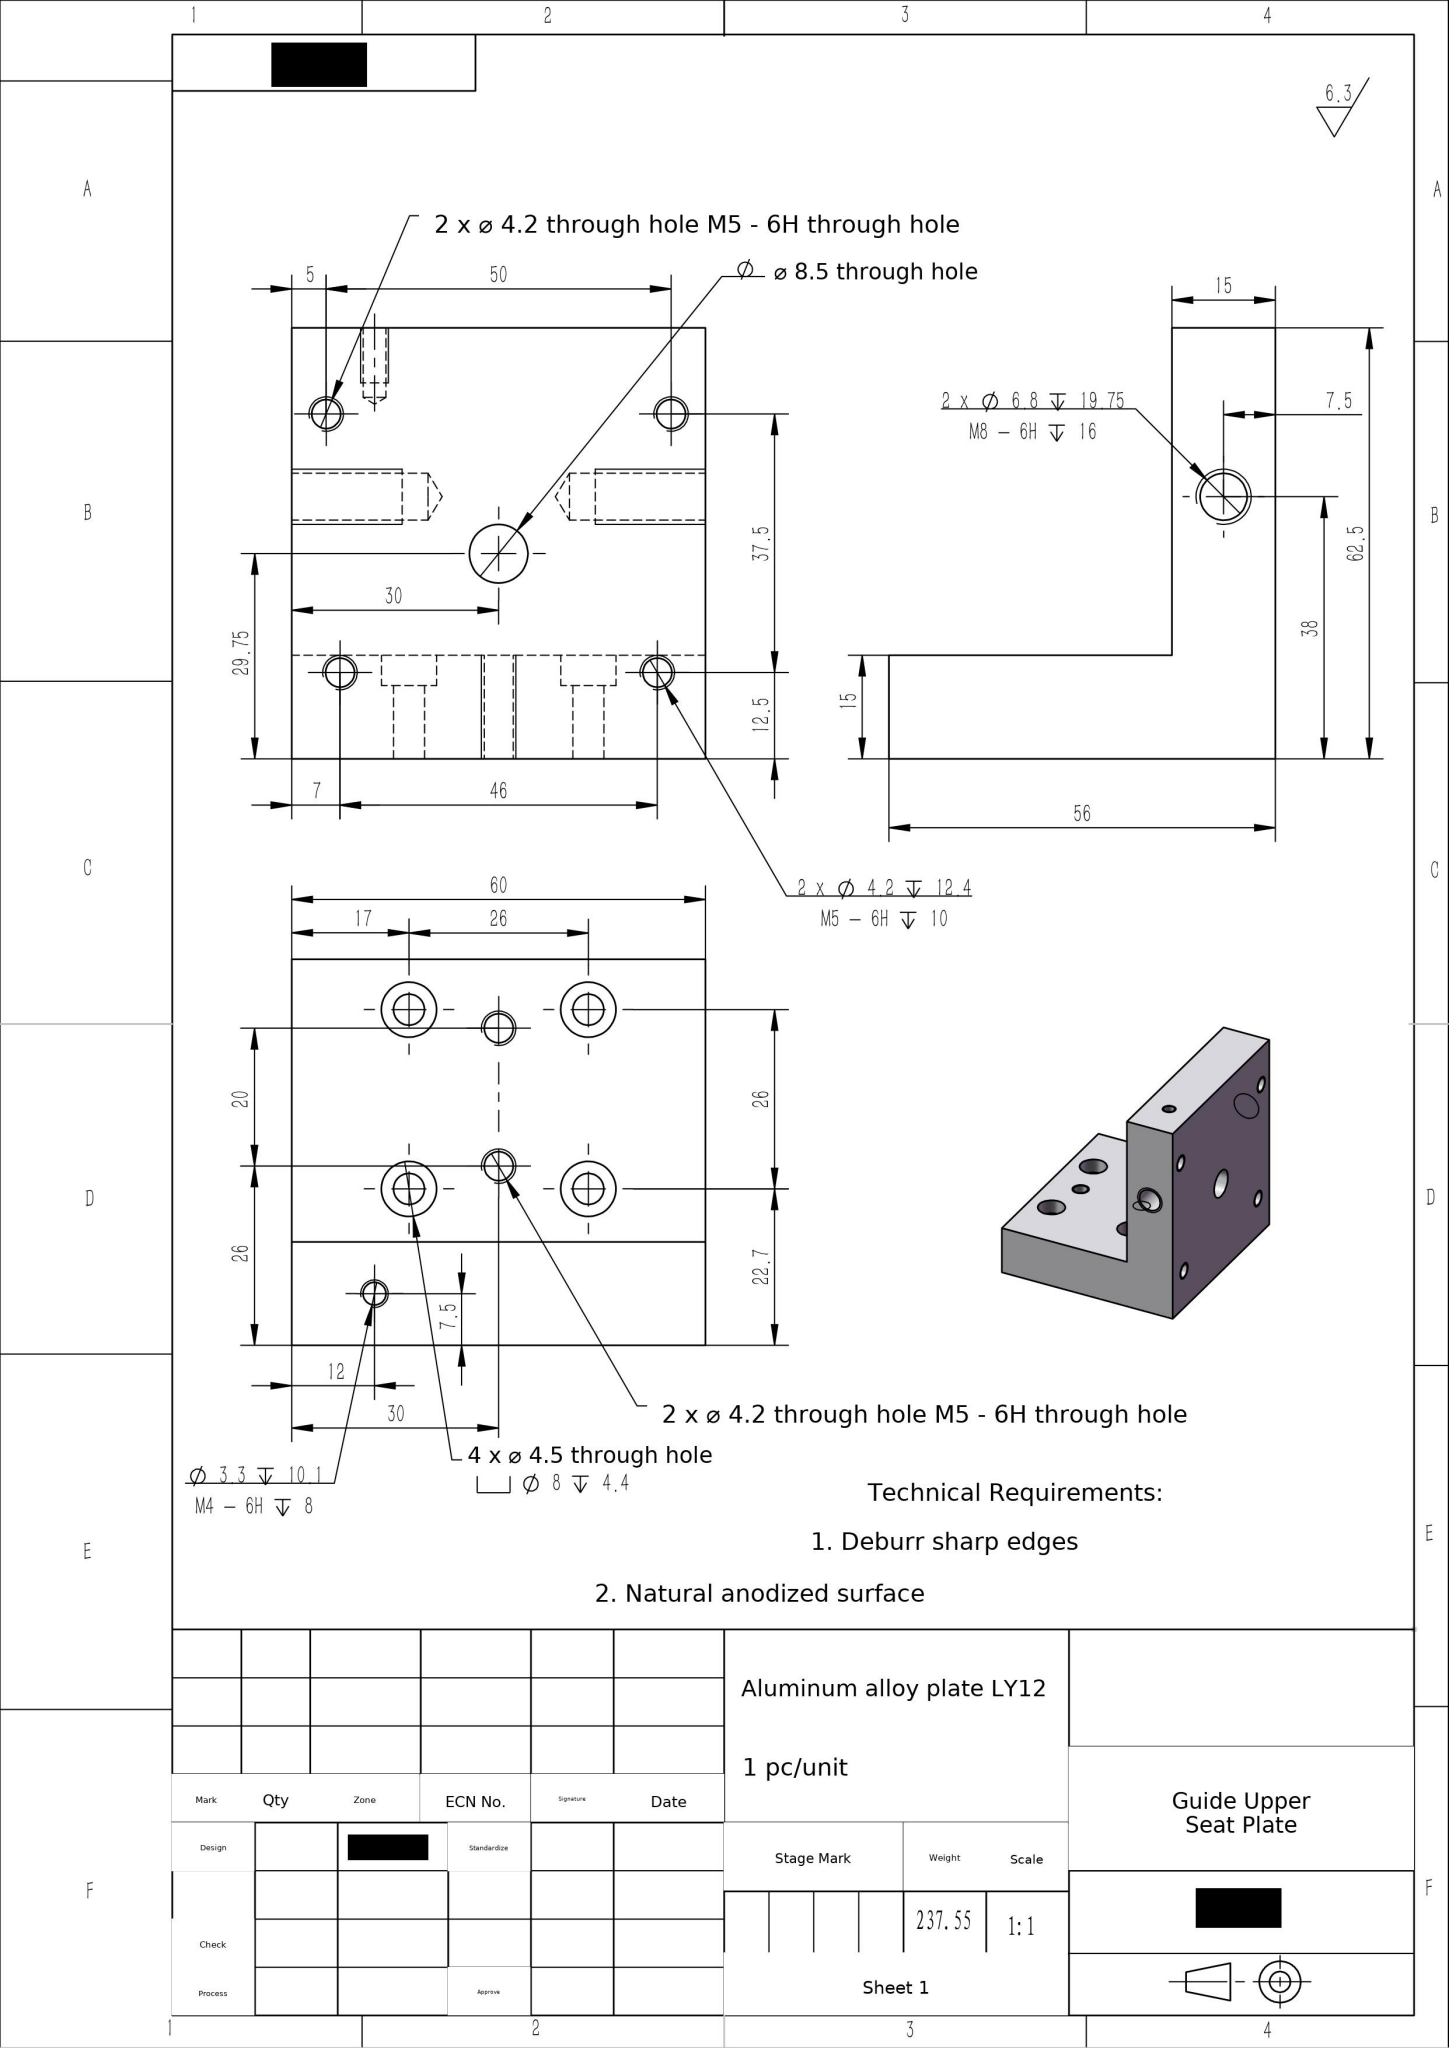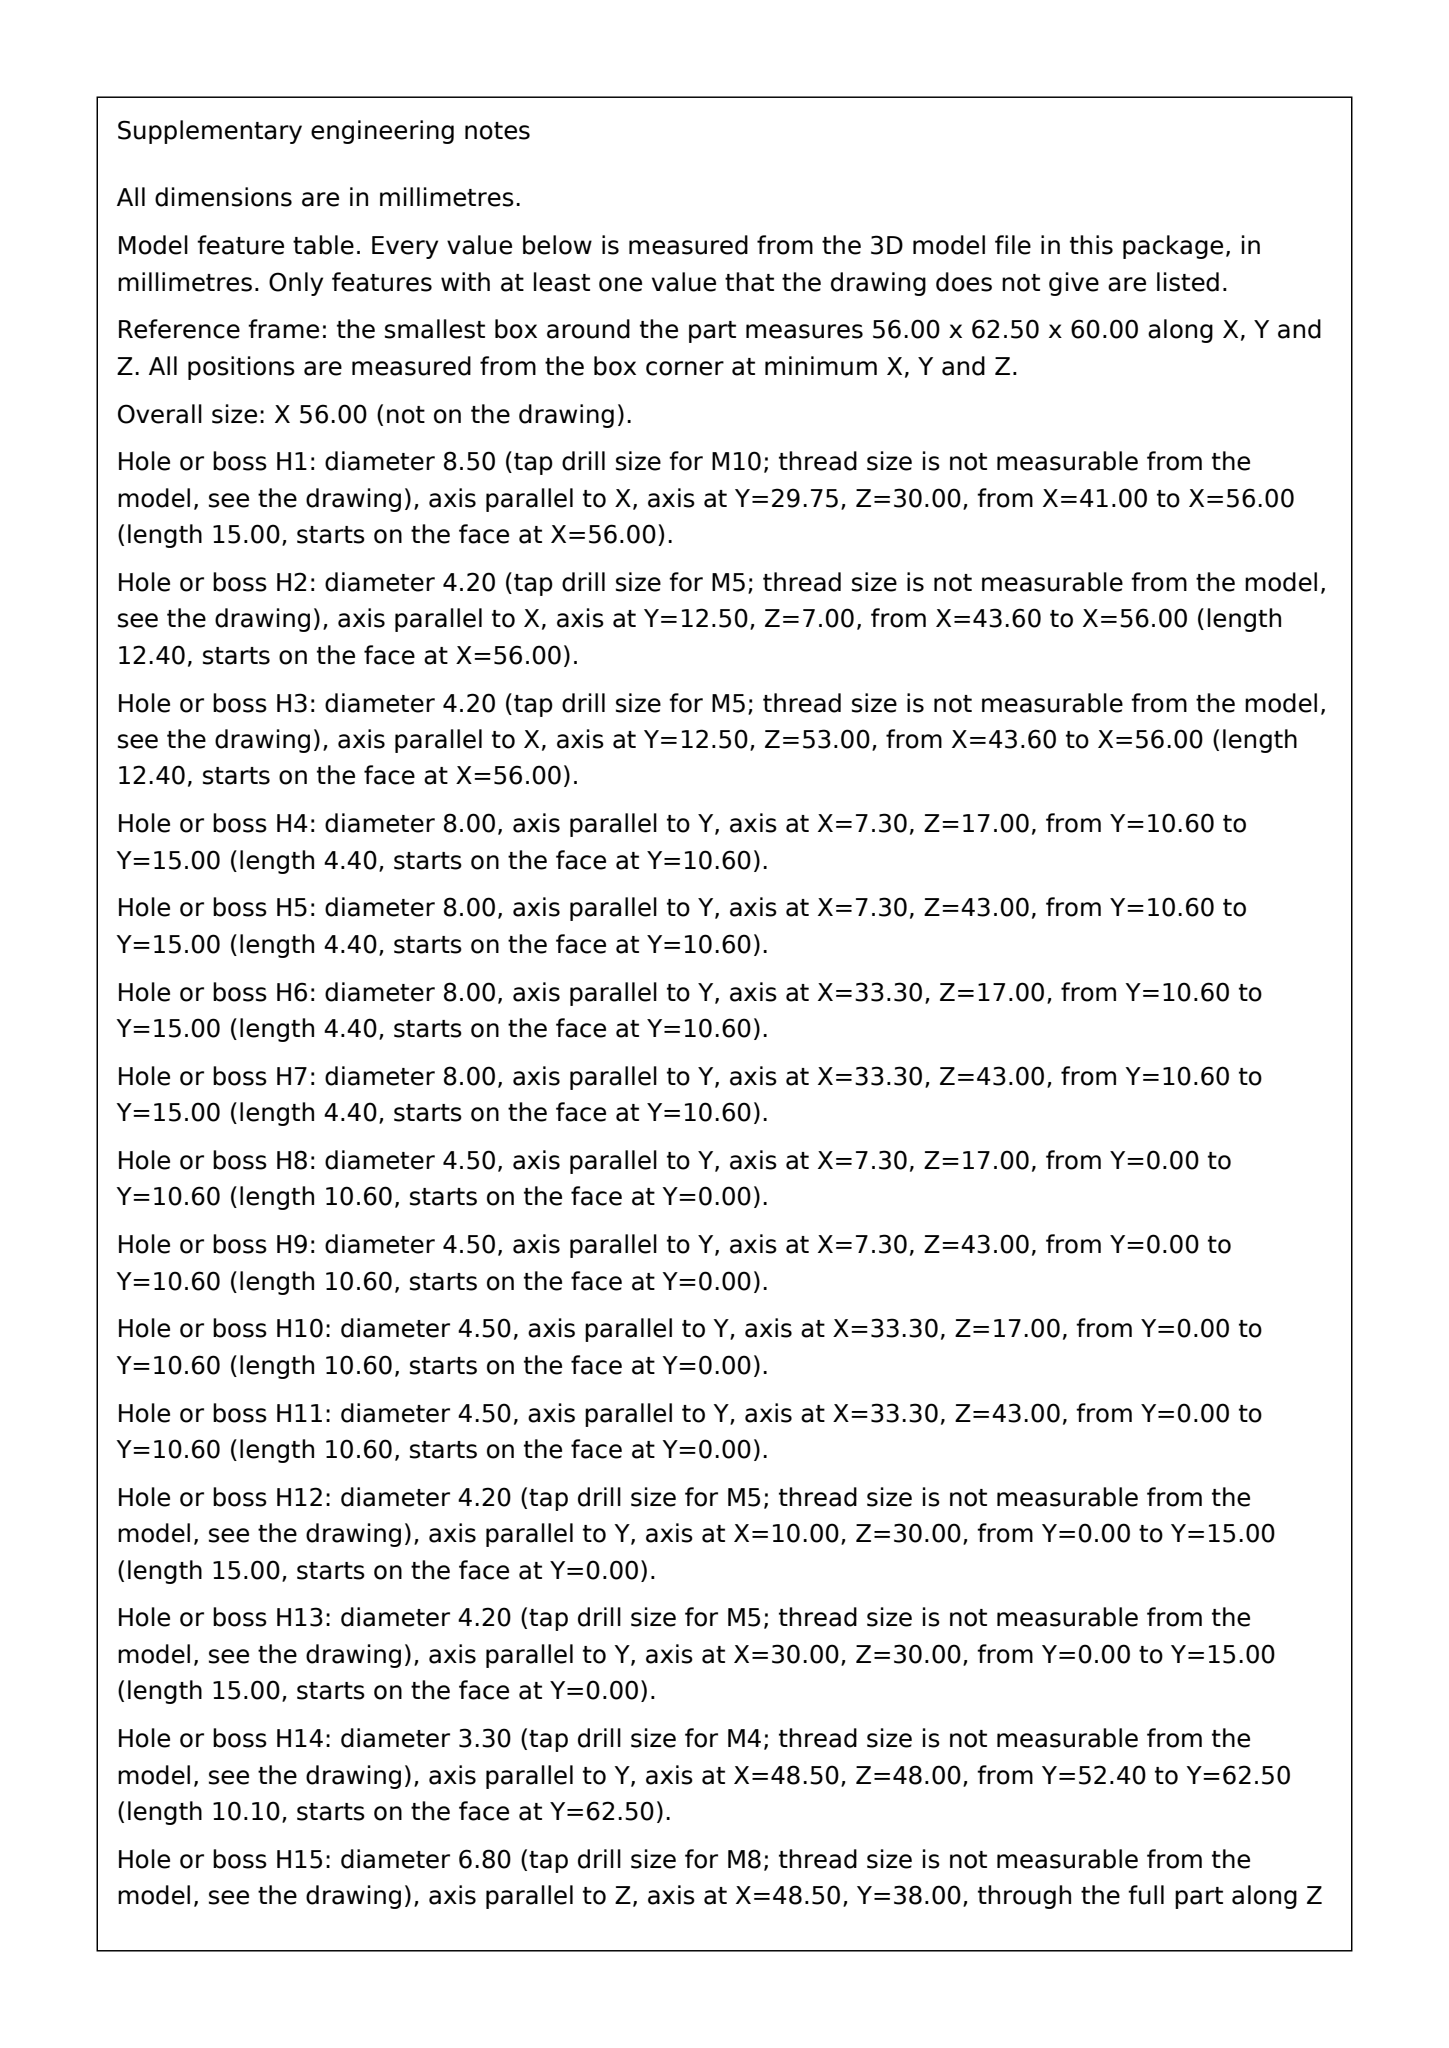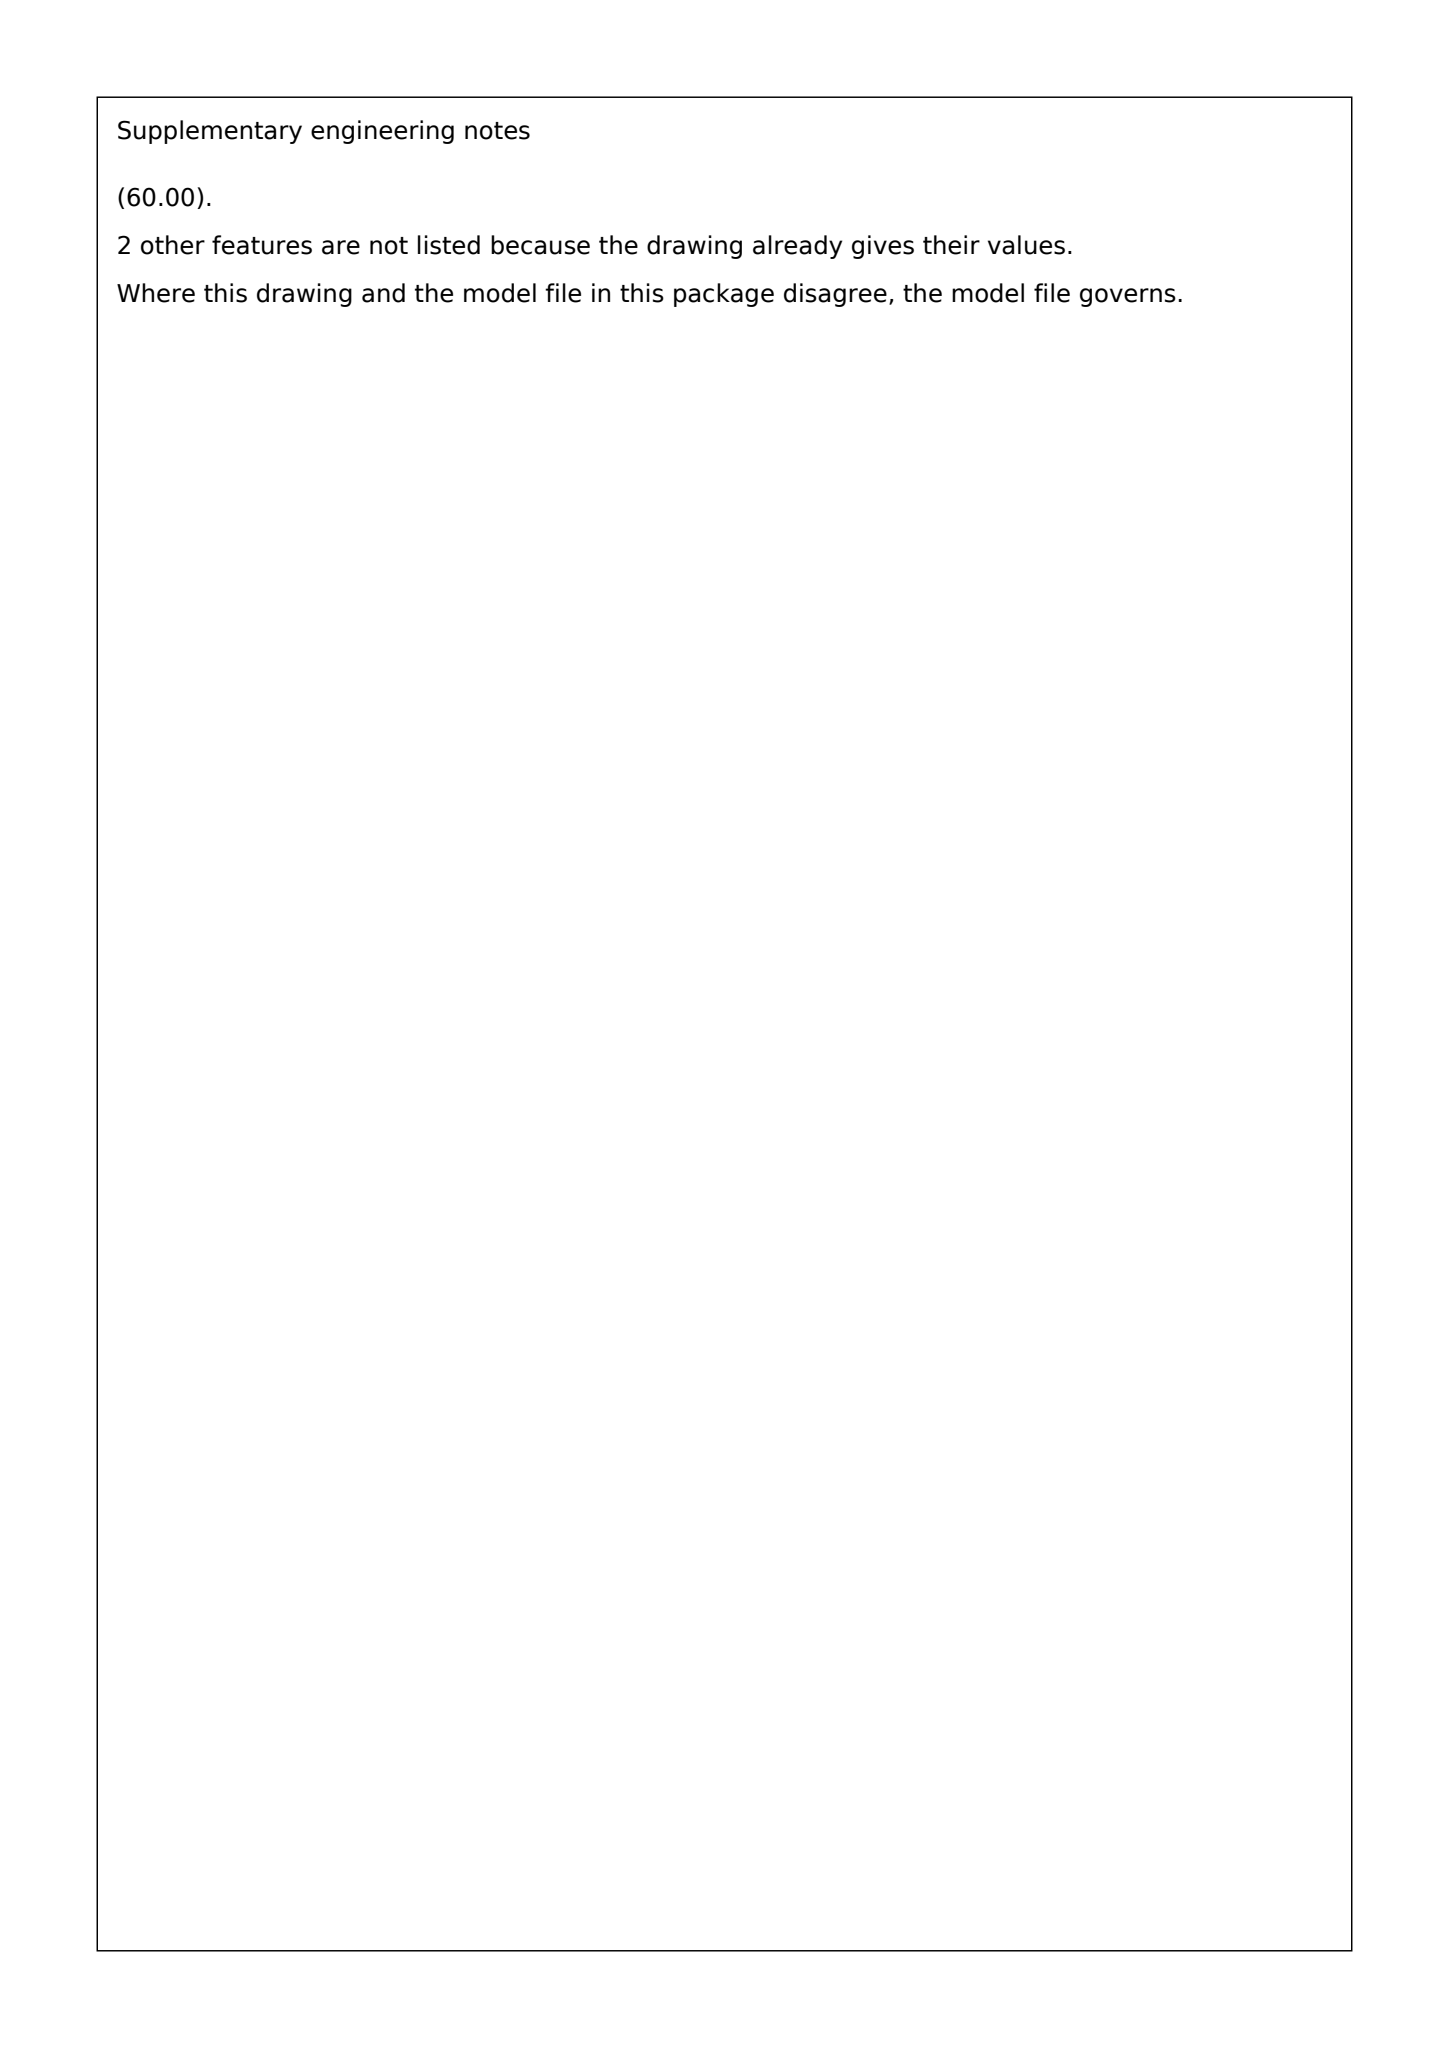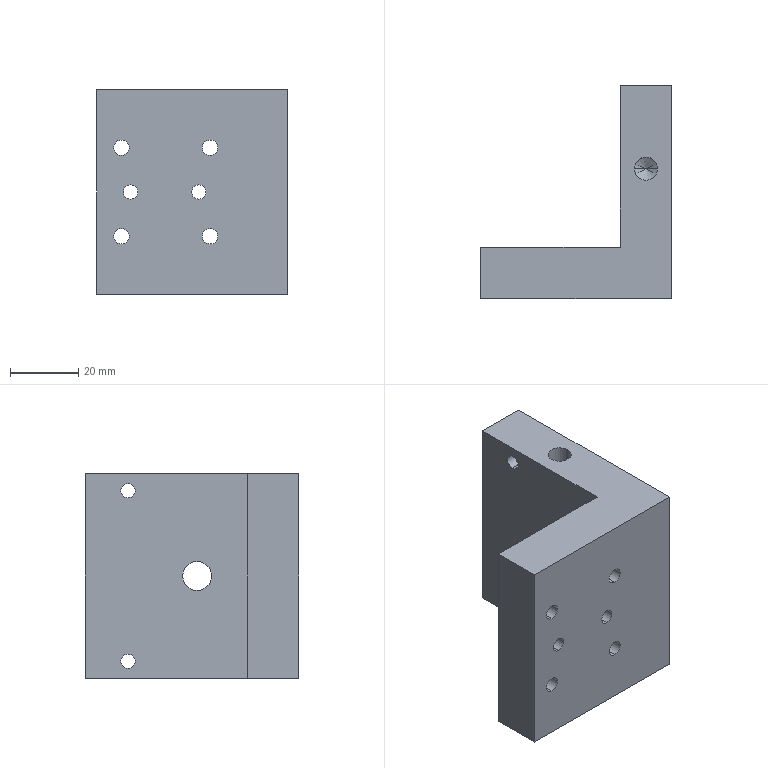Part | SolidWorks | mm | material Aluminum alloy plate LY12 | 1 solid | 58 faces | box 56 x 62.5 x 60 mm | volume 87980 mm3 | cylinder 36 | plane 12 | cone 10 | commonest cylinder face diameters 4.2 x12 8 x8 4.5 x8 6.8 x4 3.3 x2 8.5 x2
build123d program:
from build123d import *

# Parameters (mm, degrees)
BOSS_EXTRUDE1_DEPTH                             = 30
M4_HEX_SOCKET_HEAD_CAP_SCREW_CBORE1_D           = 4.5
M4_HEX_SOCKET_HEAD_CAP_SCREW_CBORE1_CBORE_D     = 8
M4_HEX_SOCKET_HEAD_CAP_SCREW_CBORE1_CBORE_DEPTH = 4.4
M5_TAPPED_HOLE1_D                               = 4.2
M5_TAPPED_HOLE2_D                               = 4.2
M5_TAPPED_HOLE2_DEPTH                           = 12.4
M5_TAPPED_HOLE2_TIP                             = 1.262
F_8_5_8_5_DIAMETER_HOLE1_D                      = 8.5
M5_TAPPED_HOLE4_D                               = 4.2
M4_TAPPED_HOLE1_D                               = 3.3
M4_TAPPED_HOLE1_DEPTH                           = 10.1
M4_TAPPED_HOLE1_TIP                             = 0.9914


with BuildPart() as part:
    # Sketch1 → Boss-Extrude1 (new, symmetric)
    with BuildSketch(Plane.XY):
        Polygon((0, 0), (0, 62.5), (-15, 62.5), (-15, 15), (-56, 15), (-56, 0), align=None)
    extrude(amount=BOSS_EXTRUDE1_DEPTH, both=True)

    # M4 Hex Socket Head Cap Screw CBORE1 (through all)
    with Locations(Plane(origin=(0, 15, 0), x_dir=(1, 0, 0), z_dir=(0, 1, 0))):
        with Locations((-48.7, -13), (-22.7, -13), (-22.7, 13), (-48.7, 13)):
            CounterBoreHole(M4_HEX_SOCKET_HEAD_CAP_SCREW_CBORE1_D / 2, M4_HEX_SOCKET_HEAD_CAP_SCREW_CBORE1_CBORE_D / 2, M4_HEX_SOCKET_HEAD_CAP_SCREW_CBORE1_CBORE_DEPTH)

    # Sketch5 → M8 Tapped Hole1 (revolve, cut)
    with BuildSketch(Plane(origin=(-7.5, 38, -30), x_dir=(0, 1, 0), z_dir=(1, 0, 0))):
        Polygon((0, 0), (0, 21.793), (3.4, 19.75), (3.4, 0), align=None)
    m8_tapped_hole1 = revolve(axis=Axis((-7.5, 38, -36.35), (0, 0, 1)), mode=Mode.SUBTRACT)

    # M5 Tapped Hole1 (through all)
    with Locations(Plane(origin=(0, 0, 0), x_dir=(0, 0, -1), z_dir=(1, 0, 0))):
        with Locations((-25, 50), (25, 50)):
            Hole(M5_TAPPED_HOLE1_D / 2)

    # M5 Tapped Hole2
    with Locations(Plane(origin=(0, 0, 0), x_dir=(0, 0, -1), z_dir=(1, 0, 0))):
        with Locations((-23, 12.5), (23, 12.5)):
            Hole(M5_TAPPED_HOLE2_D / 2, depth=M5_TAPPED_HOLE2_DEPTH)
            with Locations((0, 0, -(M5_TAPPED_HOLE2_DEPTH + M5_TAPPED_HOLE2_TIP / 2))):  # 118° drill point
                Cone(0, M5_TAPPED_HOLE2_D / 2, M5_TAPPED_HOLE2_TIP, mode=Mode.SUBTRACT)

    # Mirror1: M8 Tapped Hole1 across plane
    add(m8_tapped_hole1.mirror(Plane.XY), mode=Mode.SUBTRACT)

    # 8.5 _8.5_ Diameter Hole1 (through all)
    with Locations(Plane(origin=(0, 0, 0), x_dir=(0, 0, -1), z_dir=(1, 0, 0))):
        with Locations((0, 29.75)):
            Hole(F_8_5_8_5_DIAMETER_HOLE1_D / 2)

    # M5 Tapped Hole4 (through all)
    with Locations(Plane(origin=(0, 15, 0), x_dir=(1, 0, 0), z_dir=(0, 1, 0))):
        with Locations((-26, 0), (-46, 0)):
            Hole(M5_TAPPED_HOLE4_D / 2)

    # M4 Tapped Hole1
    with Locations(Plane(origin=(0, 62.5, 0), x_dir=(1, 0, 0), z_dir=(0, 1, 0))):
        with Locations((-7.5, -18)):
            Hole(M4_TAPPED_HOLE1_D / 2, depth=M4_TAPPED_HOLE1_DEPTH)
            with Locations((0, 0, -(M4_TAPPED_HOLE1_DEPTH + M4_TAPPED_HOLE1_TIP / 2))):  # 118° drill point
                Cone(0, M4_TAPPED_HOLE1_D / 2, M4_TAPPED_HOLE1_TIP, mode=Mode.SUBTRACT)


solid = part.part